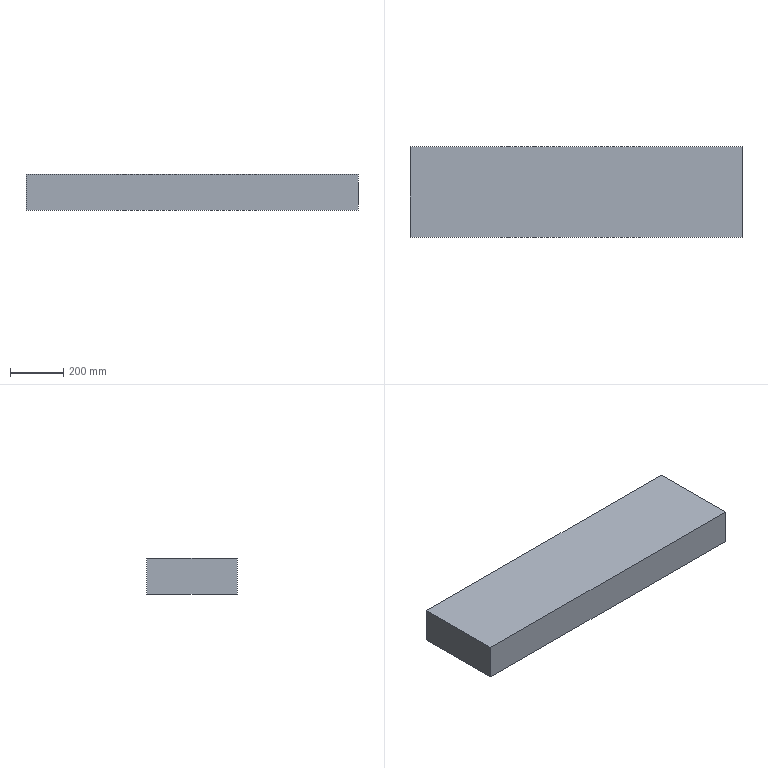Component | NX | CARTON_19 | 1 solid | 13 faces | box 1245 x 340 x 135 mm | volume 6201750 mm3 | plane 13
STEP:
#1=CARTESIAN_POINT('',(0.,0.,0.));
#2=DIRECTION('',(0.,0.,1.));
#3=DIRECTION('',(1.,0.,0.));
#4=AXIS2_PLACEMENT_3D('',#1,#2,#3);
#5=CARTESIAN_POINT('',(622.5,175.,0.));
#6=VERTEX_POINT('',#5);
#7=CARTESIAN_POINT('',(622.5,515.,0.));
#8=VERTEX_POINT('',#7);
#9=CARTESIAN_POINT('',(622.5,345.,0.));
#10=DIRECTION('',(0.,1.,0.));
#11=VECTOR('',#10,1.);
#12=LINE('',#9,#11);
#13=CARTESIAN_POINT('',(622.5,345.,0.));
#14=DIRECTION('',(1.,0.,0.));
#15=DIRECTION('',(0.,0.,-1.));
#16=AXIS2_PLACEMENT_3D('',#13,#14,#15);
#17=PLANE('',#16);
#18=CARTESIAN_POINT('',(0.,0.));
#19=DIRECTION('',(0.,1.));
#20=VECTOR('',#19,1.);
#21=LINE('',#18,#20);
#22=(GEOMETRIC_REPRESENTATION_CONTEXT(2)PARAMETRIC_REPRESENTATION_CONTEXT()REPRESENTATION_CONTEXT('',''));
#23=DEFINITIONAL_REPRESENTATION('',(#21),#22);
#24=PCURVE('',#17,#23);
#25=CARTESIAN_POINT('',(0.,345.,0.));
#26=DIRECTION('',(0.,0.,-1.));
#27=DIRECTION('',(-1.,0.,0.));
#28=AXIS2_PLACEMENT_3D('',#25,#26,#27);
#29=PLANE('',#28);
#30=CARTESIAN_POINT('',(-622.5,0.));
#31=DIRECTION('',(0.,1.));
#32=VECTOR('',#31,1.);
#33=LINE('',#30,#32);
#34=(GEOMETRIC_REPRESENTATION_CONTEXT(2)PARAMETRIC_REPRESENTATION_CONTEXT()REPRESENTATION_CONTEXT('',''));
#35=DEFINITIONAL_REPRESENTATION('',(#33),#34);
#36=PCURVE('',#29,#35);
#37=SURFACE_CURVE('',#12,(#24,#36),.PCURVE_S1.);
#38=EDGE_CURVE('',#6,#8,#37,.T.);
#39=ORIENTED_EDGE('',*,*,#38,.T.);
#40=CARTESIAN_POINT('',(622.5,515.,135.));
#41=VERTEX_POINT('',#40);
#42=CARTESIAN_POINT('',(622.5,515.,0.));
#43=DIRECTION('',(0.,0.,1.));
#44=VECTOR('',#43,1.);
#45=LINE('',#42,#44);
#46=CARTESIAN_POINT('',(0.,170.));
#47=DIRECTION('',(-1.,0.));
#48=VECTOR('',#47,1.);
#49=LINE('',#46,#48);
#50=(GEOMETRIC_REPRESENTATION_CONTEXT(2)PARAMETRIC_REPRESENTATION_CONTEXT()REPRESENTATION_CONTEXT('',''));
#51=DEFINITIONAL_REPRESENTATION('',(#49),#50);
#52=PCURVE('',#17,#51);
#53=CARTESIAN_POINT('',(0.,515.,0.));
#54=DIRECTION('',(0.,1.,0.));
#55=DIRECTION('',(0.,0.,1.));
#56=AXIS2_PLACEMENT_3D('',#53,#54,#55);
#57=PLANE('',#56);
#58=CARTESIAN_POINT('',(0.,622.5));
#59=DIRECTION('',(1.,0.));
#60=VECTOR('',#59,1.);
#61=LINE('',#58,#60);
#62=(GEOMETRIC_REPRESENTATION_CONTEXT(2)PARAMETRIC_REPRESENTATION_CONTEXT()REPRESENTATION_CONTEXT('',''));
#63=DEFINITIONAL_REPRESENTATION('',(#61),#62);
#64=PCURVE('',#57,#63);
#65=SURFACE_CURVE('',#45,(#52,#64),.PCURVE_S1.);
#66=EDGE_CURVE('',#8,#41,#65,.T.);
#67=ORIENTED_EDGE('',*,*,#66,.T.);
#68=CARTESIAN_POINT('',(622.5,175.,135.));
#69=VERTEX_POINT('',#68);
#70=CARTESIAN_POINT('',(622.5,345.,135.));
#71=DIRECTION('',(0.,-1.,0.));
#72=VECTOR('',#71,1.);
#73=LINE('',#70,#72);
#74=CARTESIAN_POINT('',(-135.,0.));
#75=DIRECTION('',(0.,-1.));
#76=VECTOR('',#75,1.);
#77=LINE('',#74,#76);
#78=(GEOMETRIC_REPRESENTATION_CONTEXT(2)PARAMETRIC_REPRESENTATION_CONTEXT()REPRESENTATION_CONTEXT('',''));
#79=DEFINITIONAL_REPRESENTATION('',(#77),#78);
#80=PCURVE('',#17,#79);
#81=CARTESIAN_POINT('',(0.,345.,135.));
#82=DIRECTION('',(0.,0.,1.));
#83=DIRECTION('',(1.,0.,0.));
#84=AXIS2_PLACEMENT_3D('',#81,#82,#83);
#85=PLANE('',#84);
#86=CARTESIAN_POINT('',(622.5,0.));
#87=DIRECTION('',(0.,-1.));
#88=VECTOR('',#87,1.);
#89=LINE('',#86,#88);
#90=(GEOMETRIC_REPRESENTATION_CONTEXT(2)PARAMETRIC_REPRESENTATION_CONTEXT()REPRESENTATION_CONTEXT('',''));
#91=DEFINITIONAL_REPRESENTATION('',(#89),#90);
#92=PCURVE('',#85,#91);
#93=SURFACE_CURVE('',#73,(#80,#92),.PCURVE_S1.);
#94=EDGE_CURVE('',#41,#69,#93,.T.);
#95=ORIENTED_EDGE('',*,*,#94,.T.);
#96=CARTESIAN_POINT('',(622.5,175.,0.));
#97=DIRECTION('',(0.,0.,1.));
#98=VECTOR('',#97,1.);
#99=LINE('',#96,#98);
#100=CARTESIAN_POINT('',(0.,-170.));
#101=DIRECTION('',(-1.,0.));
#102=VECTOR('',#101,1.);
#103=LINE('',#100,#102);
#104=(GEOMETRIC_REPRESENTATION_CONTEXT(2)PARAMETRIC_REPRESENTATION_CONTEXT()REPRESENTATION_CONTEXT('',''));
#105=DEFINITIONAL_REPRESENTATION('',(#103),#104);
#106=PCURVE('',#17,#105);
#107=CARTESIAN_POINT('',(0.,175.,0.));
#108=DIRECTION('',(0.,-1.,0.));
#109=DIRECTION('',(0.,0.,-1.));
#110=AXIS2_PLACEMENT_3D('',#107,#108,#109);
#111=PLANE('',#110);
#112=CARTESIAN_POINT('',(0.,622.5));
#113=DIRECTION('',(-1.,0.));
#114=VECTOR('',#113,1.);
#115=LINE('',#112,#114);
#116=(GEOMETRIC_REPRESENTATION_CONTEXT(2)PARAMETRIC_REPRESENTATION_CONTEXT()REPRESENTATION_CONTEXT('',''));
#117=DEFINITIONAL_REPRESENTATION('',(#115),#116);
#118=PCURVE('',#111,#117);
#119=SURFACE_CURVE('',#99,(#106,#118),.PCURVE_S1.);
#120=EDGE_CURVE('',#6,#69,#119,.T.);
#121=ORIENTED_EDGE('',*,*,#120,.F.);
#122=EDGE_LOOP('',(#39,#67,#95,#121));
#123=FACE_BOUND('',#122,.T.);
#124=CARTESIAN_POINT('',(622.5,295.,105.));
#125=VERTEX_POINT('',#124);
#126=CARTESIAN_POINT('',(622.5,395.,105.));
#127=VERTEX_POINT('',#126);
#128=CARTESIAN_POINT('',(622.5,345.,105.));
#129=DIRECTION('',(0.,1.,0.));
#130=VECTOR('',#129,1.);
#131=LINE('',#128,#130);
#132=CARTESIAN_POINT('',(-105.,0.));
#133=DIRECTION('',(0.,1.));
#134=VECTOR('',#133,1.);
#135=LINE('',#132,#134);
#136=(GEOMETRIC_REPRESENTATION_CONTEXT(2)PARAMETRIC_REPRESENTATION_CONTEXT()REPRESENTATION_CONTEXT('',''));
#137=DEFINITIONAL_REPRESENTATION('',(#135),#136);
#138=PCURVE('',#17,#137);
#139=CARTESIAN_POINT('',(622.5,345.,0.));
#140=DIRECTION('',(1.,0.,0.));
#141=DIRECTION('',(0.,0.,-1.));
#142=AXIS2_PLACEMENT_3D('',#139,#140,#141);
#143=PLANE('',#142);
#144=CARTESIAN_POINT('',(-105.,0.));
#145=DIRECTION('',(0.,1.));
#146=VECTOR('',#145,1.);
#147=LINE('',#144,#146);
#148=(GEOMETRIC_REPRESENTATION_CONTEXT(2)PARAMETRIC_REPRESENTATION_CONTEXT()REPRESENTATION_CONTEXT('',''));
#149=DEFINITIONAL_REPRESENTATION('',(#147),#148);
#150=PCURVE('',#143,#149);
#151=SURFACE_CURVE('',#131,(#138,#150),.PCURVE_S1.);
#152=EDGE_CURVE('',#125,#127,#151,.T.);
#153=ORIENTED_EDGE('',*,*,#152,.T.);
#154=CARTESIAN_POINT('',(622.5,395.,25.));
#155=VERTEX_POINT('',#154);
#156=CARTESIAN_POINT('',(622.5,395.,65.));
#157=DIRECTION('',(0.,0.,-1.));
#158=VECTOR('',#157,1.);
#159=LINE('',#156,#158);
#160=CARTESIAN_POINT('',(-65.,50.));
#161=DIRECTION('',(1.,0.));
#162=VECTOR('',#161,1.);
#163=LINE('',#160,#162);
#164=(GEOMETRIC_REPRESENTATION_CONTEXT(2)PARAMETRIC_REPRESENTATION_CONTEXT()REPRESENTATION_CONTEXT('',''));
#165=DEFINITIONAL_REPRESENTATION('',(#163),#164);
#166=PCURVE('',#17,#165);
#167=CARTESIAN_POINT('',(-65.,50.));
#168=DIRECTION('',(1.,0.));
#169=VECTOR('',#168,1.);
#170=LINE('',#167,#169);
#171=(GEOMETRIC_REPRESENTATION_CONTEXT(2)PARAMETRIC_REPRESENTATION_CONTEXT()REPRESENTATION_CONTEXT('',''));
#172=DEFINITIONAL_REPRESENTATION('',(#170),#171);
#173=PCURVE('',#143,#172);
#174=SURFACE_CURVE('',#159,(#166,#173),.PCURVE_S1.);
#175=EDGE_CURVE('',#127,#155,#174,.T.);
#176=ORIENTED_EDGE('',*,*,#175,.T.);
#177=CARTESIAN_POINT('',(622.5,295.,25.));
#178=VERTEX_POINT('',#177);
#179=CARTESIAN_POINT('',(622.5,345.,25.));
#180=DIRECTION('',(0.,-1.,0.));
#181=VECTOR('',#180,1.);
#182=LINE('',#179,#181);
#183=CARTESIAN_POINT('',(-25.,0.));
#184=DIRECTION('',(0.,-1.));
#185=VECTOR('',#184,1.);
#186=LINE('',#183,#185);
#187=(GEOMETRIC_REPRESENTATION_CONTEXT(2)PARAMETRIC_REPRESENTATION_CONTEXT()REPRESENTATION_CONTEXT('',''));
#188=DEFINITIONAL_REPRESENTATION('',(#186),#187);
#189=PCURVE('',#17,#188);
#190=CARTESIAN_POINT('',(-25.,0.));
#191=DIRECTION('',(0.,-1.));
#192=VECTOR('',#191,1.);
#193=LINE('',#190,#192);
#194=(GEOMETRIC_REPRESENTATION_CONTEXT(2)PARAMETRIC_REPRESENTATION_CONTEXT()REPRESENTATION_CONTEXT('',''));
#195=DEFINITIONAL_REPRESENTATION('',(#193),#194);
#196=PCURVE('',#143,#195);
#197=SURFACE_CURVE('',#182,(#189,#196),.PCURVE_S1.);
#198=EDGE_CURVE('',#155,#178,#197,.T.);
#199=ORIENTED_EDGE('',*,*,#198,.T.);
#200=CARTESIAN_POINT('',(622.5,295.,65.));
#201=DIRECTION('',(0.,0.,1.));
#202=VECTOR('',#201,1.);
#203=LINE('',#200,#202);
#204=CARTESIAN_POINT('',(-65.,-50.));
#205=DIRECTION('',(-1.,0.));
#206=VECTOR('',#205,1.);
#207=LINE('',#204,#206);
#208=(GEOMETRIC_REPRESENTATION_CONTEXT(2)PARAMETRIC_REPRESENTATION_CONTEXT()REPRESENTATION_CONTEXT('',''));
#209=DEFINITIONAL_REPRESENTATION('',(#207),#208);
#210=PCURVE('',#17,#209);
#211=CARTESIAN_POINT('',(-65.,-50.));
#212=DIRECTION('',(-1.,0.));
#213=VECTOR('',#212,1.);
#214=LINE('',#211,#213);
#215=(GEOMETRIC_REPRESENTATION_CONTEXT(2)PARAMETRIC_REPRESENTATION_CONTEXT()REPRESENTATION_CONTEXT('',''));
#216=DEFINITIONAL_REPRESENTATION('',(#214),#215);
#217=PCURVE('',#143,#216);
#218=SURFACE_CURVE('',#203,(#210,#217),.PCURVE_S1.);
#219=EDGE_CURVE('',#178,#125,#218,.T.);
#220=ORIENTED_EDGE('',*,*,#219,.T.);
#221=EDGE_LOOP('',(#153,#176,#199,#220));
#222=FACE_BOUND('',#221,.T.);
#223=ADVANCED_FACE('',(#123,#222),#17,.T.);
#224=CARTESIAN_POINT('',(-622.5,175.,135.));
#225=VERTEX_POINT('',#224);
#226=CARTESIAN_POINT('',(0.,175.,135.));
#227=DIRECTION('',(-1.,0.,0.));
#228=VECTOR('',#227,1.);
#229=LINE('',#226,#228);
#230=CARTESIAN_POINT('',(0.,-170.));
#231=DIRECTION('',(-1.,0.));
#232=VECTOR('',#231,1.);
#233=LINE('',#230,#232);
#234=(GEOMETRIC_REPRESENTATION_CONTEXT(2)PARAMETRIC_REPRESENTATION_CONTEXT()REPRESENTATION_CONTEXT('',''));
#235=DEFINITIONAL_REPRESENTATION('',(#233),#234);
#236=PCURVE('',#85,#235);
#237=CARTESIAN_POINT('',(-135.,0.));
#238=DIRECTION('',(0.,-1.));
#239=VECTOR('',#238,1.);
#240=LINE('',#237,#239);
#241=(GEOMETRIC_REPRESENTATION_CONTEXT(2)PARAMETRIC_REPRESENTATION_CONTEXT()REPRESENTATION_CONTEXT('',''));
#242=DEFINITIONAL_REPRESENTATION('',(#240),#241);
#243=PCURVE('',#111,#242);
#244=SURFACE_CURVE('',#229,(#236,#243),.PCURVE_S1.);
#245=EDGE_CURVE('',#69,#225,#244,.T.);
#246=ORIENTED_EDGE('',*,*,#245,.F.);
#247=ORIENTED_EDGE('',*,*,#94,.F.);
#248=CARTESIAN_POINT('',(-622.5,515.,135.));
#249=VERTEX_POINT('',#248);
#250=CARTESIAN_POINT('',(0.,515.,135.));
#251=DIRECTION('',(1.,0.,0.));
#252=VECTOR('',#251,1.);
#253=LINE('',#250,#252);
#254=CARTESIAN_POINT('',(0.,170.));
#255=DIRECTION('',(1.,0.));
#256=VECTOR('',#255,1.);
#257=LINE('',#254,#256);
#258=(GEOMETRIC_REPRESENTATION_CONTEXT(2)PARAMETRIC_REPRESENTATION_CONTEXT()REPRESENTATION_CONTEXT('',''));
#259=DEFINITIONAL_REPRESENTATION('',(#257),#258);
#260=PCURVE('',#85,#259);
#261=CARTESIAN_POINT('',(135.,0.));
#262=DIRECTION('',(0.,1.));
#263=VECTOR('',#262,1.);
#264=LINE('',#261,#263);
#265=(GEOMETRIC_REPRESENTATION_CONTEXT(2)PARAMETRIC_REPRESENTATION_CONTEXT()REPRESENTATION_CONTEXT('',''));
#266=DEFINITIONAL_REPRESENTATION('',(#264),#265);
#267=PCURVE('',#57,#266);
#268=SURFACE_CURVE('',#253,(#260,#267),.PCURVE_S1.);
#269=EDGE_CURVE('',#249,#41,#268,.T.);
#270=ORIENTED_EDGE('',*,*,#269,.F.);
#271=CARTESIAN_POINT('',(-622.5,345.,135.));
#272=DIRECTION('',(0.,1.,0.));
#273=VECTOR('',#272,1.);
#274=LINE('',#271,#273);
#275=CARTESIAN_POINT('',(-622.5,0.));
#276=DIRECTION('',(0.,1.));
#277=VECTOR('',#276,1.);
#278=LINE('',#275,#277);
#279=(GEOMETRIC_REPRESENTATION_CONTEXT(2)PARAMETRIC_REPRESENTATION_CONTEXT()REPRESENTATION_CONTEXT('',''));
#280=DEFINITIONAL_REPRESENTATION('',(#278),#279);
#281=PCURVE('',#85,#280);
#282=CARTESIAN_POINT('',(-622.5,345.,0.));
#283=DIRECTION('',(-1.,0.,0.));
#284=DIRECTION('',(0.,0.,1.));
#285=AXIS2_PLACEMENT_3D('',#282,#283,#284);
#286=PLANE('',#285);
#287=CARTESIAN_POINT('',(135.,0.));
#288=DIRECTION('',(0.,1.));
#289=VECTOR('',#288,1.);
#290=LINE('',#287,#289);
#291=(GEOMETRIC_REPRESENTATION_CONTEXT(2)PARAMETRIC_REPRESENTATION_CONTEXT()REPRESENTATION_CONTEXT('',''));
#292=DEFINITIONAL_REPRESENTATION('',(#290),#291);
#293=PCURVE('',#286,#292);
#294=SURFACE_CURVE('',#274,(#281,#293),.PCURVE_S1.);
#295=EDGE_CURVE('',#225,#249,#294,.T.);
#296=ORIENTED_EDGE('',*,*,#295,.F.);
#297=EDGE_LOOP('',(#246,#247,#270,#296));
#298=FACE_BOUND('',#297,.T.);
#299=ADVANCED_FACE('',(#298),#85,.T.);
#300=ORIENTED_EDGE('',*,*,#120,.T.);
#301=ORIENTED_EDGE('',*,*,#245,.T.);
#302=CARTESIAN_POINT('',(-622.5,175.,0.));
#303=VERTEX_POINT('',#302);
#304=CARTESIAN_POINT('',(-622.5,175.,0.));
#305=DIRECTION('',(0.,0.,1.));
#306=VECTOR('',#305,1.);
#307=LINE('',#304,#306);
#308=CARTESIAN_POINT('',(0.,-622.5));
#309=DIRECTION('',(-1.,0.));
#310=VECTOR('',#309,1.);
#311=LINE('',#308,#310);
#312=(GEOMETRIC_REPRESENTATION_CONTEXT(2)PARAMETRIC_REPRESENTATION_CONTEXT()REPRESENTATION_CONTEXT('',''));
#313=DEFINITIONAL_REPRESENTATION('',(#311),#312);
#314=PCURVE('',#111,#313);
#315=CARTESIAN_POINT('',(0.,-170.));
#316=DIRECTION('',(1.,0.));
#317=VECTOR('',#316,1.);
#318=LINE('',#315,#317);
#319=(GEOMETRIC_REPRESENTATION_CONTEXT(2)PARAMETRIC_REPRESENTATION_CONTEXT()REPRESENTATION_CONTEXT('',''));
#320=DEFINITIONAL_REPRESENTATION('',(#318),#319);
#321=PCURVE('',#286,#320);
#322=SURFACE_CURVE('',#307,(#314,#321),.PCURVE_S1.);
#323=EDGE_CURVE('',#303,#225,#322,.T.);
#324=ORIENTED_EDGE('',*,*,#323,.F.);
#325=CARTESIAN_POINT('',(0.,175.,0.));
#326=DIRECTION('',(1.,0.,0.));
#327=VECTOR('',#326,1.);
#328=LINE('',#325,#327);
#329=CARTESIAN_POINT('',(0.,0.));
#330=DIRECTION('',(0.,1.));
#331=VECTOR('',#330,1.);
#332=LINE('',#329,#331);
#333=(GEOMETRIC_REPRESENTATION_CONTEXT(2)PARAMETRIC_REPRESENTATION_CONTEXT()REPRESENTATION_CONTEXT('',''));
#334=DEFINITIONAL_REPRESENTATION('',(#332),#333);
#335=PCURVE('',#111,#334);
#336=CARTESIAN_POINT('',(0.,-170.));
#337=DIRECTION('',(-1.,0.));
#338=VECTOR('',#337,1.);
#339=LINE('',#336,#338);
#340=(GEOMETRIC_REPRESENTATION_CONTEXT(2)PARAMETRIC_REPRESENTATION_CONTEXT()REPRESENTATION_CONTEXT('',''));
#341=DEFINITIONAL_REPRESENTATION('',(#339),#340);
#342=PCURVE('',#29,#341);
#343=SURFACE_CURVE('',#328,(#335,#342),.PCURVE_S1.);
#344=EDGE_CURVE('',#303,#6,#343,.T.);
#345=ORIENTED_EDGE('',*,*,#344,.T.);
#346=EDGE_LOOP('',(#300,#301,#324,#345));
#347=FACE_BOUND('',#346,.T.);
#348=ADVANCED_FACE('',(#347),#111,.T.);
#349=ORIENTED_EDGE('',*,*,#323,.T.);
#350=ORIENTED_EDGE('',*,*,#295,.T.);
#351=CARTESIAN_POINT('',(-622.5,515.,0.));
#352=VERTEX_POINT('',#351);
#353=CARTESIAN_POINT('',(-622.5,515.,0.));
#354=DIRECTION('',(0.,0.,1.));
#355=VECTOR('',#354,1.);
#356=LINE('',#353,#355);
#357=CARTESIAN_POINT('',(0.,170.));
#358=DIRECTION('',(1.,0.));
#359=VECTOR('',#358,1.);
#360=LINE('',#357,#359);
#361=(GEOMETRIC_REPRESENTATION_CONTEXT(2)PARAMETRIC_REPRESENTATION_CONTEXT()REPRESENTATION_CONTEXT('',''));
#362=DEFINITIONAL_REPRESENTATION('',(#360),#361);
#363=PCURVE('',#286,#362);
#364=CARTESIAN_POINT('',(0.,-622.5));
#365=DIRECTION('',(1.,0.));
#366=VECTOR('',#365,1.);
#367=LINE('',#364,#366);
#368=(GEOMETRIC_REPRESENTATION_CONTEXT(2)PARAMETRIC_REPRESENTATION_CONTEXT()REPRESENTATION_CONTEXT('',''));
#369=DEFINITIONAL_REPRESENTATION('',(#367),#368);
#370=PCURVE('',#57,#369);
#371=SURFACE_CURVE('',#356,(#363,#370),.PCURVE_S1.);
#372=EDGE_CURVE('',#352,#249,#371,.T.);
#373=ORIENTED_EDGE('',*,*,#372,.F.);
#374=CARTESIAN_POINT('',(-622.5,345.,0.));
#375=DIRECTION('',(0.,-1.,0.));
#376=VECTOR('',#375,1.);
#377=LINE('',#374,#376);
#378=CARTESIAN_POINT('',(0.,0.));
#379=DIRECTION('',(0.,-1.));
#380=VECTOR('',#379,1.);
#381=LINE('',#378,#380);
#382=(GEOMETRIC_REPRESENTATION_CONTEXT(2)PARAMETRIC_REPRESENTATION_CONTEXT()REPRESENTATION_CONTEXT('',''));
#383=DEFINITIONAL_REPRESENTATION('',(#381),#382);
#384=PCURVE('',#286,#383);
#385=CARTESIAN_POINT('',(622.5,0.));
#386=DIRECTION('',(0.,-1.));
#387=VECTOR('',#386,1.);
#388=LINE('',#385,#387);
#389=(GEOMETRIC_REPRESENTATION_CONTEXT(2)PARAMETRIC_REPRESENTATION_CONTEXT()REPRESENTATION_CONTEXT('',''));
#390=DEFINITIONAL_REPRESENTATION('',(#388),#389);
#391=PCURVE('',#29,#390);
#392=SURFACE_CURVE('',#377,(#384,#391),.PCURVE_S1.);
#393=EDGE_CURVE('',#352,#303,#392,.T.);
#394=ORIENTED_EDGE('',*,*,#393,.T.);
#395=EDGE_LOOP('',(#349,#350,#373,#394));
#396=FACE_BOUND('',#395,.T.);
#397=ADVANCED_FACE('',(#396),#286,.T.);
#398=ORIENTED_EDGE('',*,*,#372,.T.);
#399=ORIENTED_EDGE('',*,*,#269,.T.);
#400=ORIENTED_EDGE('',*,*,#66,.F.);
#401=CARTESIAN_POINT('',(0.,515.,0.));
#402=DIRECTION('',(-1.,0.,0.));
#403=VECTOR('',#402,1.);
#404=LINE('',#401,#403);
#405=CARTESIAN_POINT('',(0.,0.));
#406=DIRECTION('',(0.,-1.));
#407=VECTOR('',#406,1.);
#408=LINE('',#405,#407);
#409=(GEOMETRIC_REPRESENTATION_CONTEXT(2)PARAMETRIC_REPRESENTATION_CONTEXT()REPRESENTATION_CONTEXT('',''));
#410=DEFINITIONAL_REPRESENTATION('',(#408),#409);
#411=PCURVE('',#57,#410);
#412=CARTESIAN_POINT('',(0.,170.));
#413=DIRECTION('',(1.,0.));
#414=VECTOR('',#413,1.);
#415=LINE('',#412,#414);
#416=(GEOMETRIC_REPRESENTATION_CONTEXT(2)PARAMETRIC_REPRESENTATION_CONTEXT()REPRESENTATION_CONTEXT('',''));
#417=DEFINITIONAL_REPRESENTATION('',(#415),#416);
#418=PCURVE('',#29,#417);
#419=SURFACE_CURVE('',#404,(#411,#418),.PCURVE_S1.);
#420=EDGE_CURVE('',#8,#352,#419,.T.);
#421=ORIENTED_EDGE('',*,*,#420,.T.);
#422=EDGE_LOOP('',(#398,#399,#400,#421));
#423=FACE_BOUND('',#422,.T.);
#424=ADVANCED_FACE('',(#423),#57,.T.);
#425=ORIENTED_EDGE('',*,*,#38,.F.);
#426=ORIENTED_EDGE('',*,*,#344,.F.);
#427=ORIENTED_EDGE('',*,*,#393,.F.);
#428=ORIENTED_EDGE('',*,*,#420,.F.);
#429=EDGE_LOOP('',(#425,#426,#427,#428));
#430=FACE_BOUND('',#429,.T.);
#431=ADVANCED_FACE('',(#430),#29,.T.);
#432=ORIENTED_EDGE('',*,*,#175,.F.);
#433=ORIENTED_EDGE('',*,*,#152,.F.);
#434=ORIENTED_EDGE('',*,*,#219,.F.);
#435=ORIENTED_EDGE('',*,*,#198,.F.);
#436=EDGE_LOOP('',(#432,#433,#434,#435));
#437=FACE_BOUND('',#436,.T.);
#438=ADVANCED_FACE('',(#437),#143,.T.);
#439=CLOSED_SHELL('',(#223,#299,#348,#397,#424,#431,#438));
#440=CARTESIAN_POINT('',(617.5,180.,130.));
#441=VERTEX_POINT('',#440);
#442=CARTESIAN_POINT('',(-617.5,180.,130.));
#443=VERTEX_POINT('',#442);
#444=CARTESIAN_POINT('',(0.,180.,130.));
#445=DIRECTION('',(-1.,0.,0.));
#446=VECTOR('',#445,1.);
#447=LINE('',#444,#446);
#448=CARTESIAN_POINT('',(0.,345.,130.));
#449=DIRECTION('',(0.,0.,1.));
#450=DIRECTION('',(1.,0.,0.));
#451=AXIS2_PLACEMENT_3D('',#448,#449,#450);
#452=PLANE('',#451);
#453=CARTESIAN_POINT('',(0.,-165.));
#454=DIRECTION('',(-1.,0.));
#455=VECTOR('',#454,1.);
#456=LINE('',#453,#455);
#457=(GEOMETRIC_REPRESENTATION_CONTEXT(2)PARAMETRIC_REPRESENTATION_CONTEXT()REPRESENTATION_CONTEXT('',''));
#458=DEFINITIONAL_REPRESENTATION('',(#456),#457);
#459=PCURVE('',#452,#458);
#460=CARTESIAN_POINT('',(0.,180.,0.));
#461=DIRECTION('',(0.,-1.,0.));
#462=DIRECTION('',(0.,0.,-1.));
#463=AXIS2_PLACEMENT_3D('',#460,#461,#462);
#464=PLANE('',#463);
#465=CARTESIAN_POINT('',(-130.,0.));
#466=DIRECTION('',(0.,-1.));
#467=VECTOR('',#466,1.);
#468=LINE('',#465,#467);
#469=(GEOMETRIC_REPRESENTATION_CONTEXT(2)PARAMETRIC_REPRESENTATION_CONTEXT()REPRESENTATION_CONTEXT('',''));
#470=DEFINITIONAL_REPRESENTATION('',(#468),#469);
#471=PCURVE('',#464,#470);
#472=SURFACE_CURVE('',#447,(#459,#471),.PCURVE_S1.);
#473=EDGE_CURVE('',#441,#443,#472,.T.);
#474=ORIENTED_EDGE('',*,*,#473,.T.);
#475=CARTESIAN_POINT('',(-617.5,510.,130.));
#476=VERTEX_POINT('',#475);
#477=CARTESIAN_POINT('',(-617.5,345.,130.));
#478=DIRECTION('',(0.,1.,0.));
#479=VECTOR('',#478,1.);
#480=LINE('',#477,#479);
#481=CARTESIAN_POINT('',(-617.5,0.));
#482=DIRECTION('',(0.,1.));
#483=VECTOR('',#482,1.);
#484=LINE('',#481,#483);
#485=(GEOMETRIC_REPRESENTATION_CONTEXT(2)PARAMETRIC_REPRESENTATION_CONTEXT()REPRESENTATION_CONTEXT('',''));
#486=DEFINITIONAL_REPRESENTATION('',(#484),#485);
#487=PCURVE('',#452,#486);
#488=CARTESIAN_POINT('',(-617.5,345.,0.));
#489=DIRECTION('',(-1.,0.,0.));
#490=DIRECTION('',(0.,0.,1.));
#491=AXIS2_PLACEMENT_3D('',#488,#489,#490);
#492=PLANE('',#491);
#493=CARTESIAN_POINT('',(130.,0.));
#494=DIRECTION('',(0.,1.));
#495=VECTOR('',#494,1.);
#496=LINE('',#493,#495);
#497=(GEOMETRIC_REPRESENTATION_CONTEXT(2)PARAMETRIC_REPRESENTATION_CONTEXT()REPRESENTATION_CONTEXT('',''));
#498=DEFINITIONAL_REPRESENTATION('',(#496),#497);
#499=PCURVE('',#492,#498);
#500=SURFACE_CURVE('',#480,(#487,#499),.PCURVE_S1.);
#501=EDGE_CURVE('',#443,#476,#500,.T.);
#502=ORIENTED_EDGE('',*,*,#501,.T.);
#503=CARTESIAN_POINT('',(617.5,510.,130.));
#504=VERTEX_POINT('',#503);
#505=CARTESIAN_POINT('',(0.,510.,130.));
#506=DIRECTION('',(1.,0.,0.));
#507=VECTOR('',#506,1.);
#508=LINE('',#505,#507);
#509=CARTESIAN_POINT('',(0.,165.));
#510=DIRECTION('',(1.,0.));
#511=VECTOR('',#510,1.);
#512=LINE('',#509,#511);
#513=(GEOMETRIC_REPRESENTATION_CONTEXT(2)PARAMETRIC_REPRESENTATION_CONTEXT()REPRESENTATION_CONTEXT('',''));
#514=DEFINITIONAL_REPRESENTATION('',(#512),#513);
#515=PCURVE('',#452,#514);
#516=CARTESIAN_POINT('',(0.,510.,0.));
#517=DIRECTION('',(0.,1.,0.));
#518=DIRECTION('',(0.,0.,1.));
#519=AXIS2_PLACEMENT_3D('',#516,#517,#518);
#520=PLANE('',#519);
#521=CARTESIAN_POINT('',(130.,0.));
#522=DIRECTION('',(0.,1.));
#523=VECTOR('',#522,1.);
#524=LINE('',#521,#523);
#525=(GEOMETRIC_REPRESENTATION_CONTEXT(2)PARAMETRIC_REPRESENTATION_CONTEXT()REPRESENTATION_CONTEXT('',''));
#526=DEFINITIONAL_REPRESENTATION('',(#524),#525);
#527=PCURVE('',#520,#526);
#528=SURFACE_CURVE('',#508,(#515,#527),.PCURVE_S1.);
#529=EDGE_CURVE('',#476,#504,#528,.T.);
#530=ORIENTED_EDGE('',*,*,#529,.T.);
#531=CARTESIAN_POINT('',(617.5,345.,130.));
#532=DIRECTION('',(0.,-1.,0.));
#533=VECTOR('',#532,1.);
#534=LINE('',#531,#533);
#535=CARTESIAN_POINT('',(617.5,0.));
#536=DIRECTION('',(0.,-1.));
#537=VECTOR('',#536,1.);
#538=LINE('',#535,#537);
#539=(GEOMETRIC_REPRESENTATION_CONTEXT(2)PARAMETRIC_REPRESENTATION_CONTEXT()REPRESENTATION_CONTEXT('',''));
#540=DEFINITIONAL_REPRESENTATION('',(#538),#539);
#541=PCURVE('',#452,#540);
#542=CARTESIAN_POINT('',(617.5,345.,0.));
#543=DIRECTION('',(1.,0.,0.));
#544=DIRECTION('',(0.,0.,-1.));
#545=AXIS2_PLACEMENT_3D('',#542,#543,#544);
#546=PLANE('',#545);
#547=CARTESIAN_POINT('',(-130.,0.));
#548=DIRECTION('',(0.,-1.));
#549=VECTOR('',#548,1.);
#550=LINE('',#547,#549);
#551=(GEOMETRIC_REPRESENTATION_CONTEXT(2)PARAMETRIC_REPRESENTATION_CONTEXT()REPRESENTATION_CONTEXT('',''));
#552=DEFINITIONAL_REPRESENTATION('',(#550),#551);
#553=PCURVE('',#546,#552);
#554=SURFACE_CURVE('',#534,(#541,#553),.PCURVE_S1.);
#555=EDGE_CURVE('',#504,#441,#554,.T.);
#556=ORIENTED_EDGE('',*,*,#555,.T.);
#557=EDGE_LOOP('',(#474,#502,#530,#556));
#558=FACE_BOUND('',#557,.F.);
#559=ADVANCED_FACE('',(#558),#452,.T.);
#560=CARTESIAN_POINT('',(617.5,180.,5.));
#561=VERTEX_POINT('',#560);
#562=CARTESIAN_POINT('',(617.5,180.,0.));
#563=DIRECTION('',(0.,0.,1.));
#564=VECTOR('',#563,1.);
#565=LINE('',#562,#564);
#566=CARTESIAN_POINT('',(0.,617.5));
#567=DIRECTION('',(-1.,0.));
#568=VECTOR('',#567,1.);
#569=LINE('',#566,#568);
#570=(GEOMETRIC_REPRESENTATION_CONTEXT(2)PARAMETRIC_REPRESENTATION_CONTEXT()REPRESENTATION_CONTEXT('',''));
#571=DEFINITIONAL_REPRESENTATION('',(#569),#570);
#572=PCURVE('',#464,#571);
#573=CARTESIAN_POINT('',(0.,-165.));
#574=DIRECTION('',(-1.,0.));
#575=VECTOR('',#574,1.);
#576=LINE('',#573,#575);
#577=(GEOMETRIC_REPRESENTATION_CONTEXT(2)PARAMETRIC_REPRESENTATION_CONTEXT()REPRESENTATION_CONTEXT('',''));
#578=DEFINITIONAL_REPRESENTATION('',(#576),#577);
#579=PCURVE('',#546,#578);
#580=SURFACE_CURVE('',#565,(#572,#579),.PCURVE_S1.);
#581=EDGE_CURVE('',#561,#441,#580,.T.);
#582=ORIENTED_EDGE('',*,*,#581,.F.);
#583=CARTESIAN_POINT('',(-617.5,180.,5.));
#584=VERTEX_POINT('',#583);
#585=CARTESIAN_POINT('',(0.,180.,5.));
#586=DIRECTION('',(1.,0.,0.));
#587=VECTOR('',#586,1.);
#588=LINE('',#585,#587);
#589=CARTESIAN_POINT('',(-5.,0.));
#590=DIRECTION('',(0.,1.));
#591=VECTOR('',#590,1.);
#592=LINE('',#589,#591);
#593=(GEOMETRIC_REPRESENTATION_CONTEXT(2)PARAMETRIC_REPRESENTATION_CONTEXT()REPRESENTATION_CONTEXT('',''));
#594=DEFINITIONAL_REPRESENTATION('',(#592),#593);
#595=PCURVE('',#464,#594);
#596=CARTESIAN_POINT('',(0.,345.,5.));
#597=DIRECTION('',(0.,0.,-1.));
#598=DIRECTION('',(-1.,0.,0.));
#599=AXIS2_PLACEMENT_3D('',#596,#597,#598);
#600=PLANE('',#599);
#601=CARTESIAN_POINT('',(0.,-165.));
#602=DIRECTION('',(-1.,0.));
#603=VECTOR('',#602,1.);
#604=LINE('',#601,#603);
#605=(GEOMETRIC_REPRESENTATION_CONTEXT(2)PARAMETRIC_REPRESENTATION_CONTEXT()REPRESENTATION_CONTEXT('',''));
#606=DEFINITIONAL_REPRESENTATION('',(#604),#605);
#607=PCURVE('',#600,#606);
#608=SURFACE_CURVE('',#588,(#595,#607),.PCURVE_S1.);
#609=EDGE_CURVE('',#584,#561,#608,.T.);
#610=ORIENTED_EDGE('',*,*,#609,.F.);
#611=CARTESIAN_POINT('',(-617.5,180.,0.));
#612=DIRECTION('',(0.,0.,1.));
#613=VECTOR('',#612,1.);
#614=LINE('',#611,#613);
#615=CARTESIAN_POINT('',(0.,-617.5));
#616=DIRECTION('',(-1.,0.));
#617=VECTOR('',#616,1.);
#618=LINE('',#615,#617);
#619=(GEOMETRIC_REPRESENTATION_CONTEXT(2)PARAMETRIC_REPRESENTATION_CONTEXT()REPRESENTATION_CONTEXT('',''));
#620=DEFINITIONAL_REPRESENTATION('',(#618),#619);
#621=PCURVE('',#464,#620);
#622=CARTESIAN_POINT('',(0.,-165.));
#623=DIRECTION('',(1.,0.));
#624=VECTOR('',#623,1.);
#625=LINE('',#622,#624);
#626=(GEOMETRIC_REPRESENTATION_CONTEXT(2)PARAMETRIC_REPRESENTATION_CONTEXT()REPRESENTATION_CONTEXT('',''));
#627=DEFINITIONAL_REPRESENTATION('',(#625),#626);
#628=PCURVE('',#492,#627);
#629=SURFACE_CURVE('',#614,(#621,#628),.PCURVE_S1.);
#630=EDGE_CURVE('',#584,#443,#629,.T.);
#631=ORIENTED_EDGE('',*,*,#630,.T.);
#632=ORIENTED_EDGE('',*,*,#473,.F.);
#633=EDGE_LOOP('',(#582,#610,#631,#632));
#634=FACE_BOUND('',#633,.F.);
#635=ADVANCED_FACE('',(#634),#464,.T.);
#636=ORIENTED_EDGE('',*,*,#630,.F.);
#637=CARTESIAN_POINT('',(-617.5,510.,5.));
#638=VERTEX_POINT('',#637);
#639=CARTESIAN_POINT('',(-617.5,345.,5.));
#640=DIRECTION('',(0.,-1.,0.));
#641=VECTOR('',#640,1.);
#642=LINE('',#639,#641);
#643=CARTESIAN_POINT('',(5.,0.));
#644=DIRECTION('',(0.,-1.));
#645=VECTOR('',#644,1.);
#646=LINE('',#643,#645);
#647=(GEOMETRIC_REPRESENTATION_CONTEXT(2)PARAMETRIC_REPRESENTATION_CONTEXT()REPRESENTATION_CONTEXT('',''));
#648=DEFINITIONAL_REPRESENTATION('',(#646),#647);
#649=PCURVE('',#492,#648);
#650=CARTESIAN_POINT('',(617.5,0.));
#651=DIRECTION('',(0.,-1.));
#652=VECTOR('',#651,1.);
#653=LINE('',#650,#652);
#654=(GEOMETRIC_REPRESENTATION_CONTEXT(2)PARAMETRIC_REPRESENTATION_CONTEXT()REPRESENTATION_CONTEXT('',''));
#655=DEFINITIONAL_REPRESENTATION('',(#653),#654);
#656=PCURVE('',#600,#655);
#657=SURFACE_CURVE('',#642,(#649,#656),.PCURVE_S1.);
#658=EDGE_CURVE('',#638,#584,#657,.T.);
#659=ORIENTED_EDGE('',*,*,#658,.F.);
#660=CARTESIAN_POINT('',(-617.5,510.,0.));
#661=DIRECTION('',(0.,0.,1.));
#662=VECTOR('',#661,1.);
#663=LINE('',#660,#662);
#664=CARTESIAN_POINT('',(0.,165.));
#665=DIRECTION('',(1.,0.));
#666=VECTOR('',#665,1.);
#667=LINE('',#664,#666);
#668=(GEOMETRIC_REPRESENTATION_CONTEXT(2)PARAMETRIC_REPRESENTATION_CONTEXT()REPRESENTATION_CONTEXT('',''));
#669=DEFINITIONAL_REPRESENTATION('',(#667),#668);
#670=PCURVE('',#492,#669);
#671=CARTESIAN_POINT('',(0.,-617.5));
#672=DIRECTION('',(1.,0.));
#673=VECTOR('',#672,1.);
#674=LINE('',#671,#673);
#675=(GEOMETRIC_REPRESENTATION_CONTEXT(2)PARAMETRIC_REPRESENTATION_CONTEXT()REPRESENTATION_CONTEXT('',''));
#676=DEFINITIONAL_REPRESENTATION('',(#674),#675);
#677=PCURVE('',#520,#676);
#678=SURFACE_CURVE('',#663,(#670,#677),.PCURVE_S1.);
#679=EDGE_CURVE('',#638,#476,#678,.T.);
#680=ORIENTED_EDGE('',*,*,#679,.T.);
#681=ORIENTED_EDGE('',*,*,#501,.F.);
#682=EDGE_LOOP('',(#636,#659,#680,#681));
#683=FACE_BOUND('',#682,.F.);
#684=ADVANCED_FACE('',(#683),#492,.T.);
#685=ORIENTED_EDGE('',*,*,#679,.F.);
#686=CARTESIAN_POINT('',(617.5,510.,5.));
#687=VERTEX_POINT('',#686);
#688=CARTESIAN_POINT('',(0.,510.,5.));
#689=DIRECTION('',(-1.,0.,0.));
#690=VECTOR('',#689,1.);
#691=LINE('',#688,#690);
#692=CARTESIAN_POINT('',(5.,0.));
#693=DIRECTION('',(0.,-1.));
#694=VECTOR('',#693,1.);
#695=LINE('',#692,#694);
#696=(GEOMETRIC_REPRESENTATION_CONTEXT(2)PARAMETRIC_REPRESENTATION_CONTEXT()REPRESENTATION_CONTEXT('',''));
#697=DEFINITIONAL_REPRESENTATION('',(#695),#696);
#698=PCURVE('',#520,#697);
#699=CARTESIAN_POINT('',(0.,165.));
#700=DIRECTION('',(1.,0.));
#701=VECTOR('',#700,1.);
#702=LINE('',#699,#701);
#703=(GEOMETRIC_REPRESENTATION_CONTEXT(2)PARAMETRIC_REPRESENTATION_CONTEXT()REPRESENTATION_CONTEXT('',''));
#704=DEFINITIONAL_REPRESENTATION('',(#702),#703);
#705=PCURVE('',#600,#704);
#706=SURFACE_CURVE('',#691,(#698,#705),.PCURVE_S1.);
#707=EDGE_CURVE('',#687,#638,#706,.T.);
#708=ORIENTED_EDGE('',*,*,#707,.F.);
#709=CARTESIAN_POINT('',(617.5,510.,0.));
#710=DIRECTION('',(0.,0.,1.));
#711=VECTOR('',#710,1.);
#712=LINE('',#709,#711);
#713=CARTESIAN_POINT('',(0.,617.5));
#714=DIRECTION('',(1.,0.));
#715=VECTOR('',#714,1.);
#716=LINE('',#713,#715);
#717=(GEOMETRIC_REPRESENTATION_CONTEXT(2)PARAMETRIC_REPRESENTATION_CONTEXT()REPRESENTATION_CONTEXT('',''));
#718=DEFINITIONAL_REPRESENTATION('',(#716),#717);
#719=PCURVE('',#520,#718);
#720=CARTESIAN_POINT('',(0.,165.));
#721=DIRECTION('',(-1.,0.));
#722=VECTOR('',#721,1.);
#723=LINE('',#720,#722);
#724=(GEOMETRIC_REPRESENTATION_CONTEXT(2)PARAMETRIC_REPRESENTATION_CONTEXT()REPRESENTATION_CONTEXT('',''));
#725=DEFINITIONAL_REPRESENTATION('',(#723),#724);
#726=PCURVE('',#546,#725);
#727=SURFACE_CURVE('',#712,(#719,#726),.PCURVE_S1.);
#728=EDGE_CURVE('',#687,#504,#727,.T.);
#729=ORIENTED_EDGE('',*,*,#728,.T.);
#730=ORIENTED_EDGE('',*,*,#529,.F.);
#731=EDGE_LOOP('',(#685,#708,#729,#730));
#732=FACE_BOUND('',#731,.F.);
#733=ADVANCED_FACE('',(#732),#520,.T.);
#734=CARTESIAN_POINT('',(617.5,345.,5.));
#735=DIRECTION('',(0.,1.,0.));
#736=VECTOR('',#735,1.);
#737=LINE('',#734,#736);
#738=CARTESIAN_POINT('',(-617.5,0.));
#739=DIRECTION('',(0.,1.));
#740=VECTOR('',#739,1.);
#741=LINE('',#738,#740);
#742=(GEOMETRIC_REPRESENTATION_CONTEXT(2)PARAMETRIC_REPRESENTATION_CONTEXT()REPRESENTATION_CONTEXT('',''));
#743=DEFINITIONAL_REPRESENTATION('',(#741),#742);
#744=PCURVE('',#600,#743);
#745=CARTESIAN_POINT('',(-5.,0.));
#746=DIRECTION('',(0.,1.));
#747=VECTOR('',#746,1.);
#748=LINE('',#745,#747);
#749=(GEOMETRIC_REPRESENTATION_CONTEXT(2)PARAMETRIC_REPRESENTATION_CONTEXT()REPRESENTATION_CONTEXT('',''));
#750=DEFINITIONAL_REPRESENTATION('',(#748),#749);
#751=PCURVE('',#546,#750);
#752=SURFACE_CURVE('',#737,(#744,#751),.PCURVE_S1.);
#753=EDGE_CURVE('',#561,#687,#752,.T.);
#754=ORIENTED_EDGE('',*,*,#753,.T.);
#755=ORIENTED_EDGE('',*,*,#707,.T.);
#756=ORIENTED_EDGE('',*,*,#658,.T.);
#757=ORIENTED_EDGE('',*,*,#609,.T.);
#758=EDGE_LOOP('',(#754,#755,#756,#757));
#759=FACE_BOUND('',#758,.F.);
#760=ADVANCED_FACE('',(#759),#600,.T.);
#761=ORIENTED_EDGE('',*,*,#753,.F.);
#762=ORIENTED_EDGE('',*,*,#581,.T.);
#763=ORIENTED_EDGE('',*,*,#555,.F.);
#764=ORIENTED_EDGE('',*,*,#728,.F.);
#765=EDGE_LOOP('',(#761,#762,#763,#764));
#766=FACE_BOUND('',#765,.F.);
#767=ADVANCED_FACE('',(#766),#546,.T.);
#768=CLOSED_SHELL('',(#559,#635,#684,#733,#760,#767));
#769=ORIENTED_CLOSED_SHELL('',*,#768,.F.);
#770=BREP_WITH_VOIDS('',#439,(#769));
#771=(LENGTH_UNIT()NAMED_UNIT(*)SI_UNIT(.MILLI.,.METRE.));
#772=UNCERTAINTY_MEASURE_WITH_UNIT(LENGTH_MEASURE(0.0000001),#771,'','');
#773=(NAMED_UNIT(*)PLANE_ANGLE_UNIT()SI_UNIT($,.RADIAN.));
#774=(NAMED_UNIT(*)SI_UNIT($,.STERADIAN.)SOLID_ANGLE_UNIT());
#775=(GEOMETRIC_REPRESENTATION_CONTEXT(3)GLOBAL_UNCERTAINTY_ASSIGNED_CONTEXT((#772))GLOBAL_UNIT_ASSIGNED_CONTEXT((#771,#773,#774))REPRESENTATION_CONTEXT('',''));
#776=ADVANCED_BREP_SHAPE_REPRESENTATION('',(#4,#770),#775);